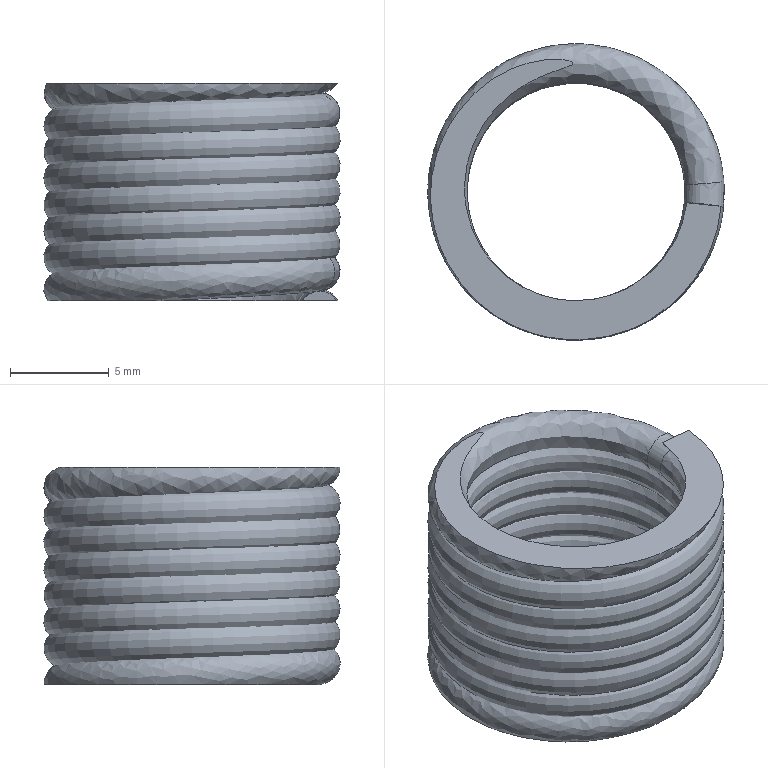Component | NX | SPRING | 1 solid | 9 faces | volume 946 mm3 | spline 5 | plane 4